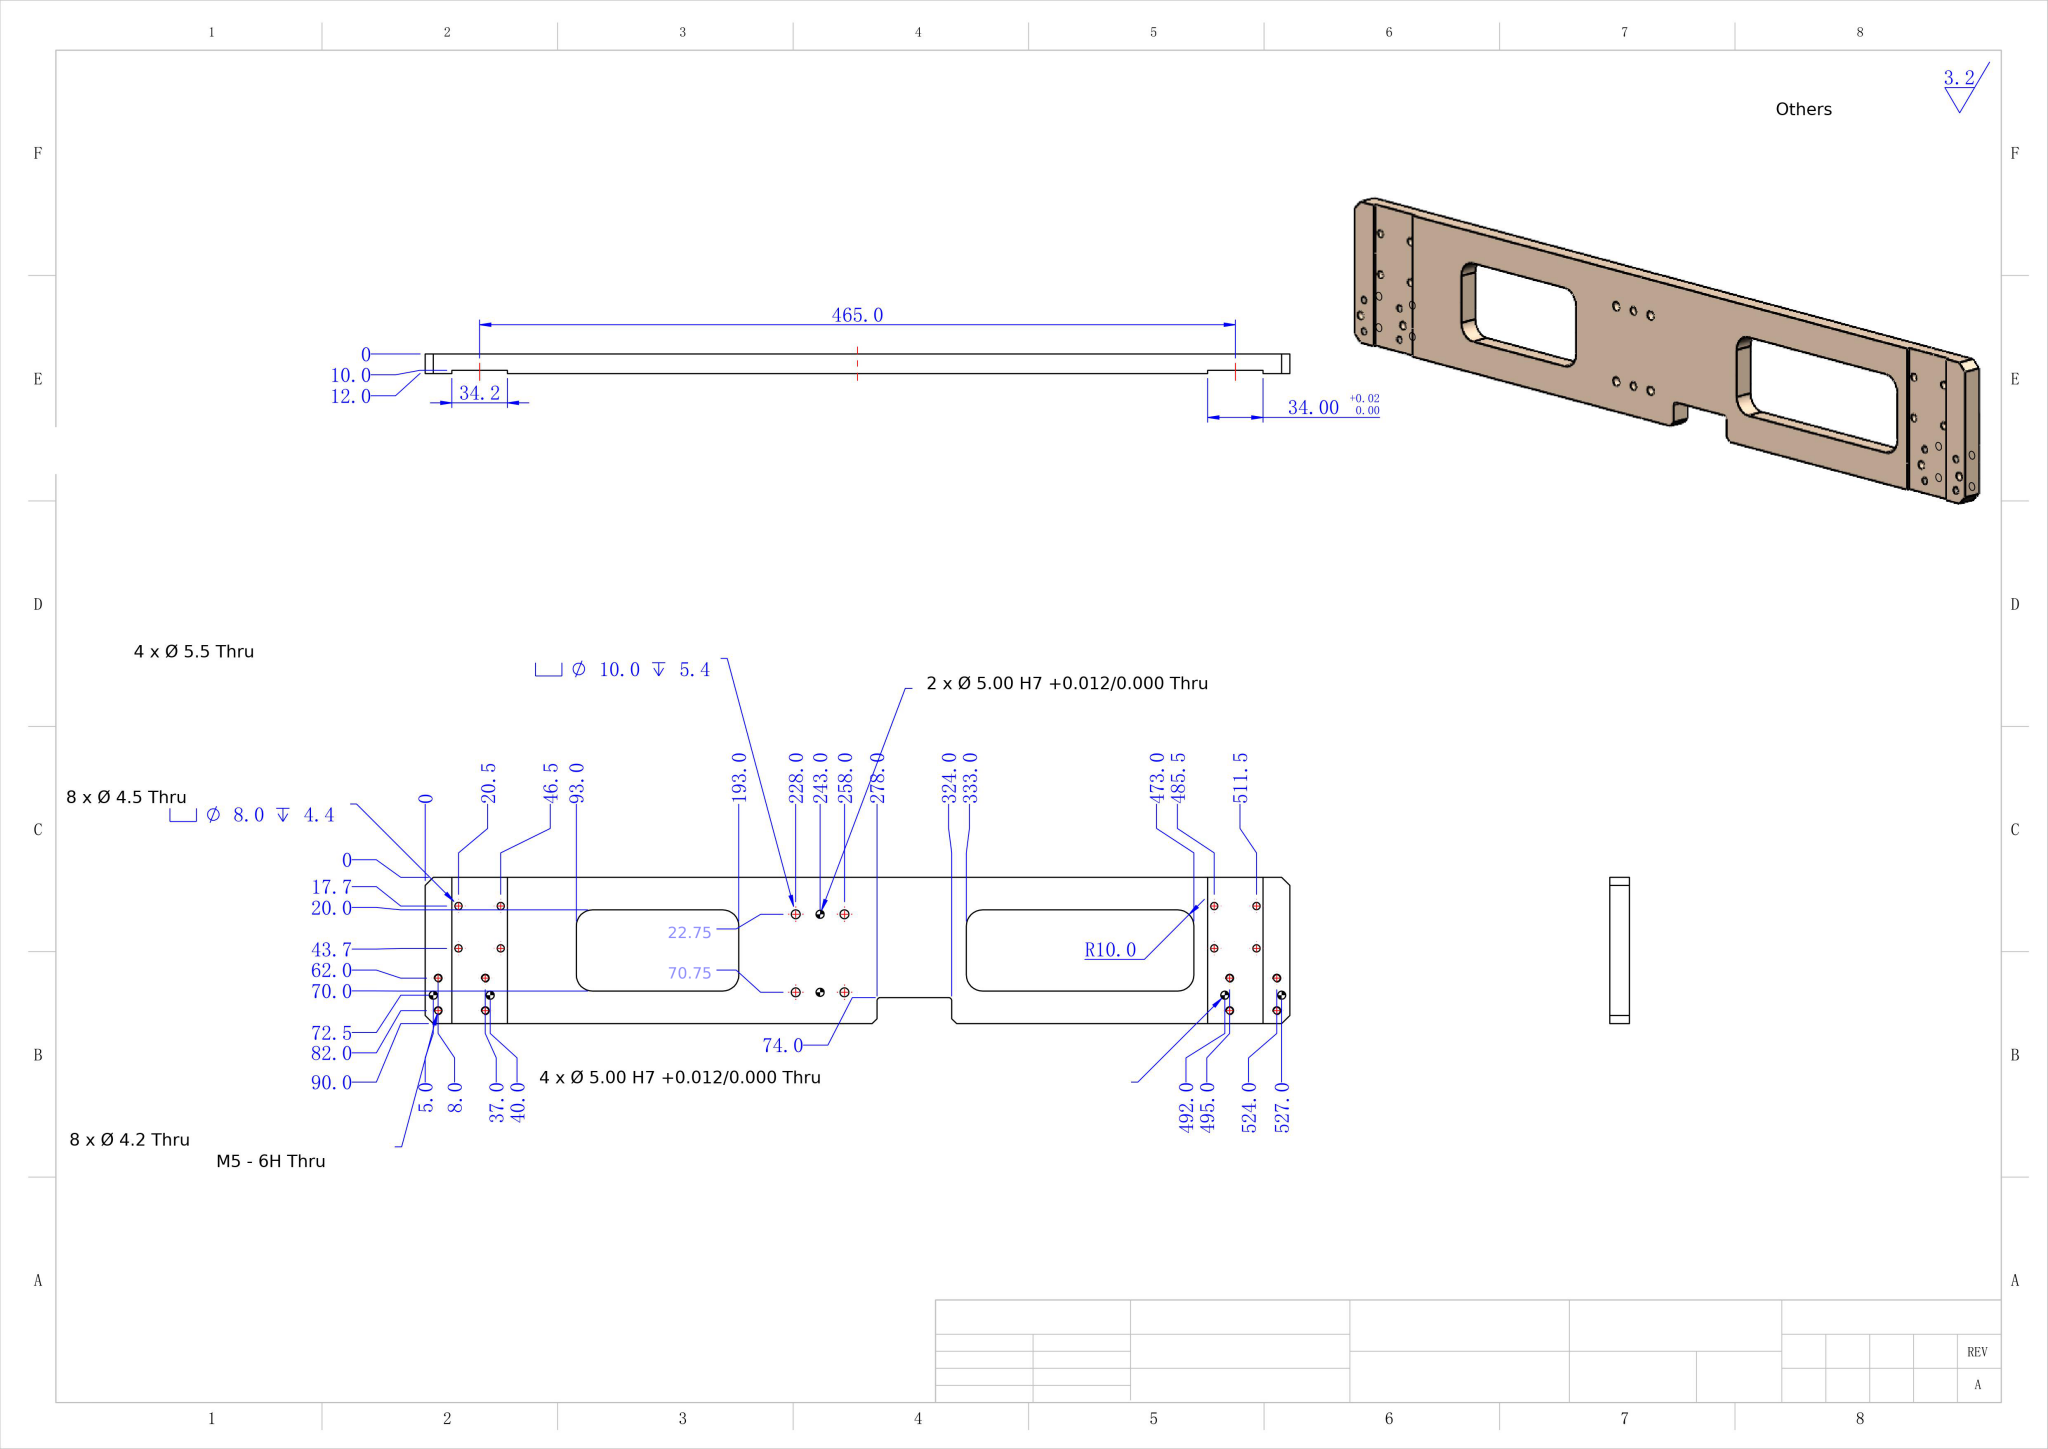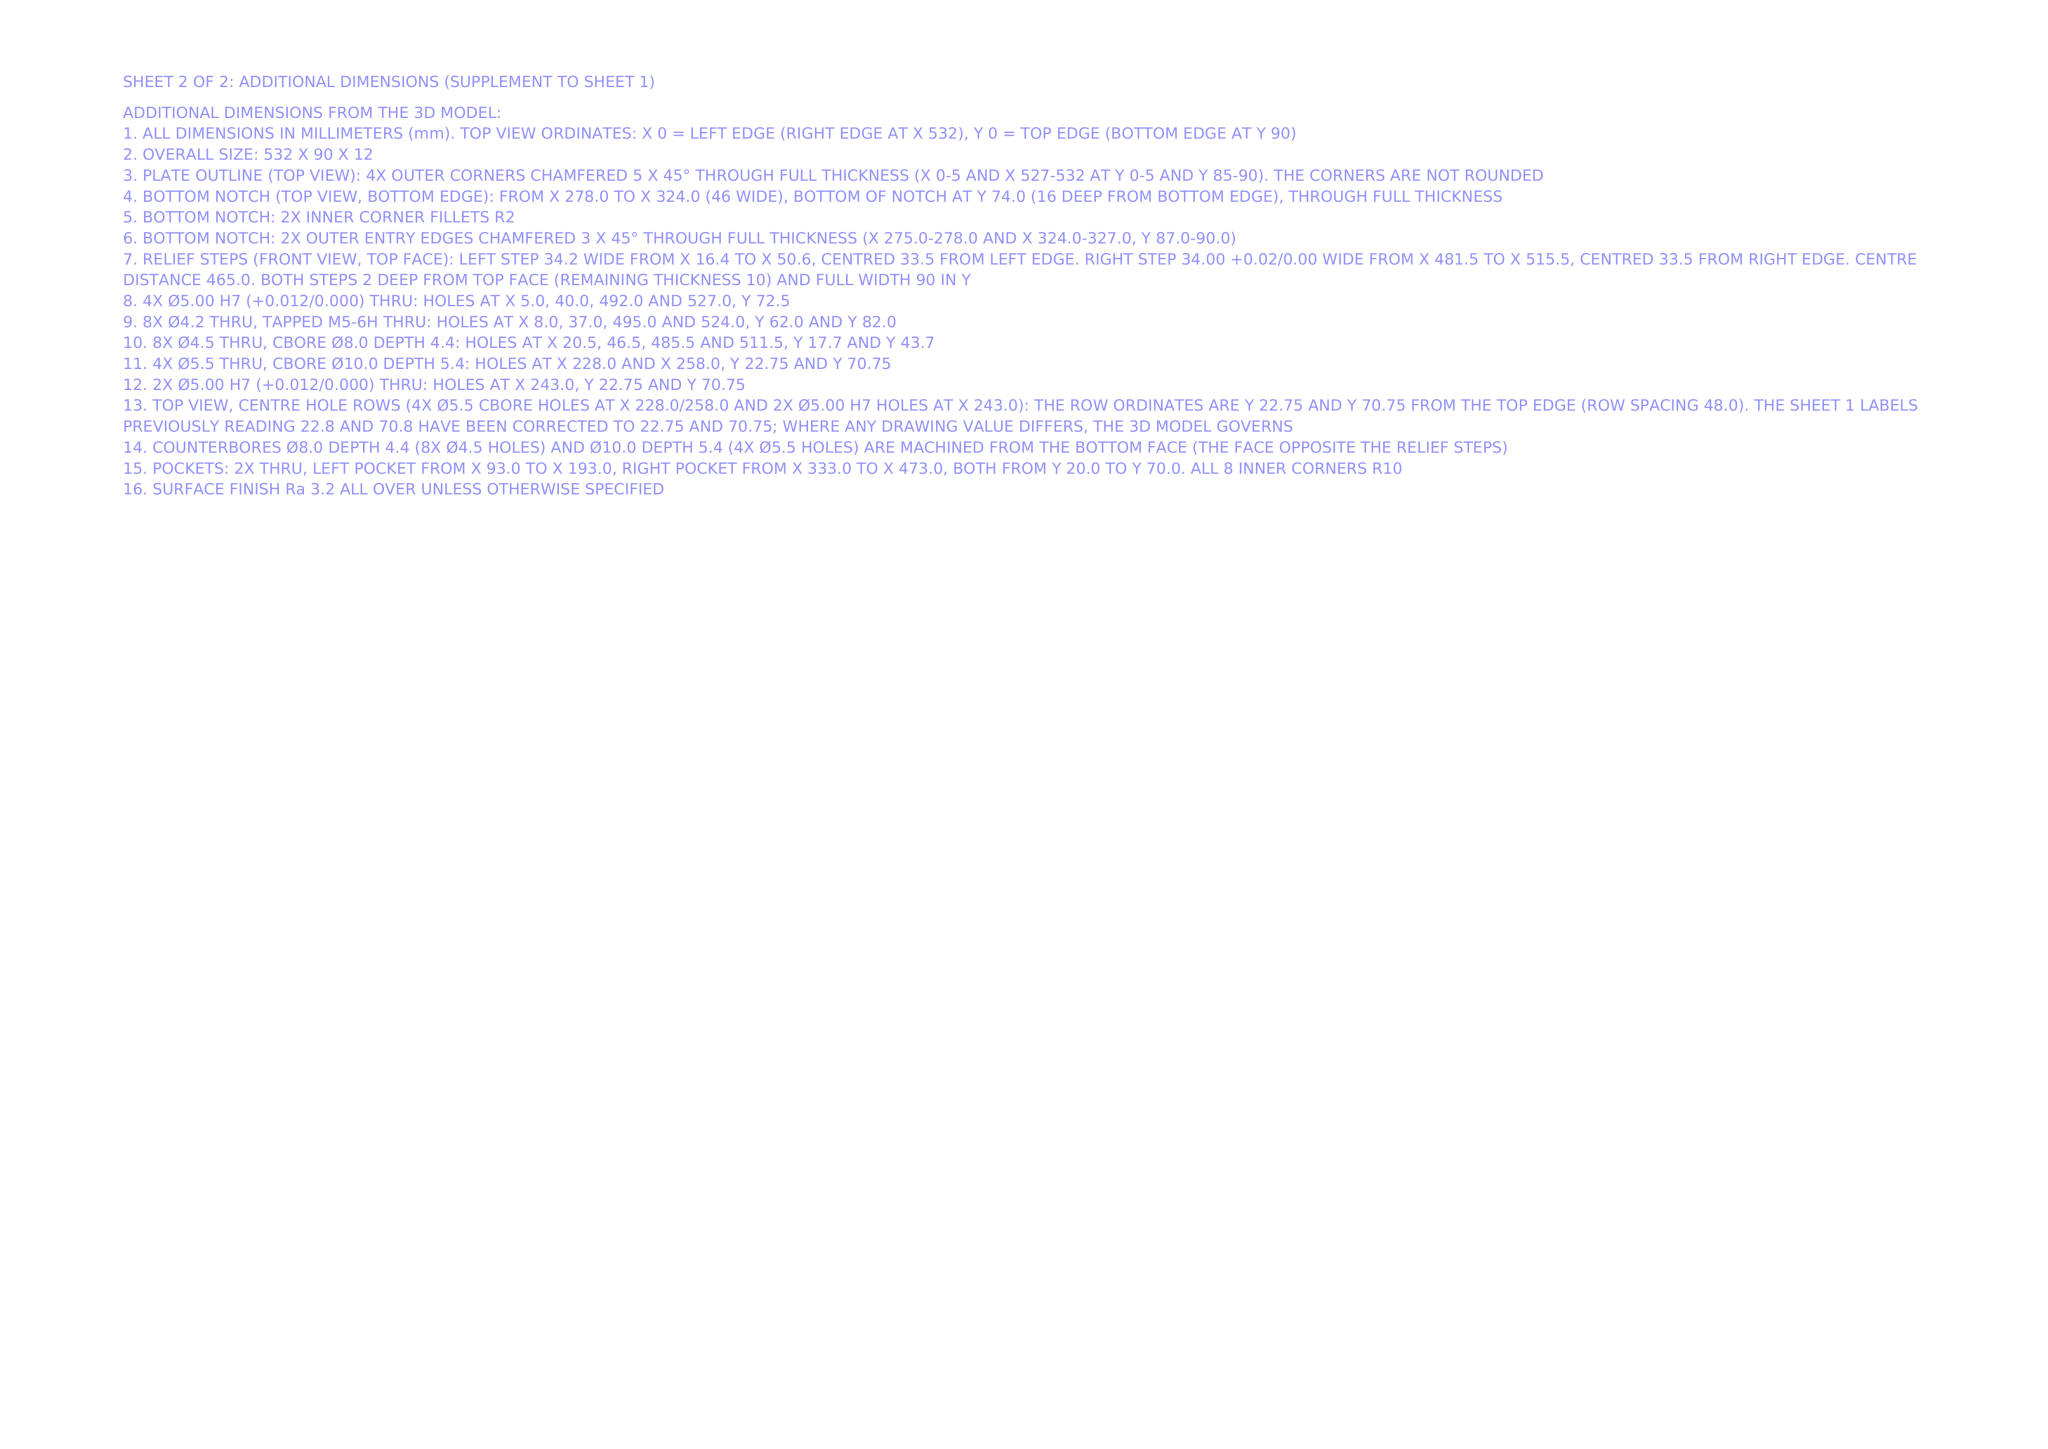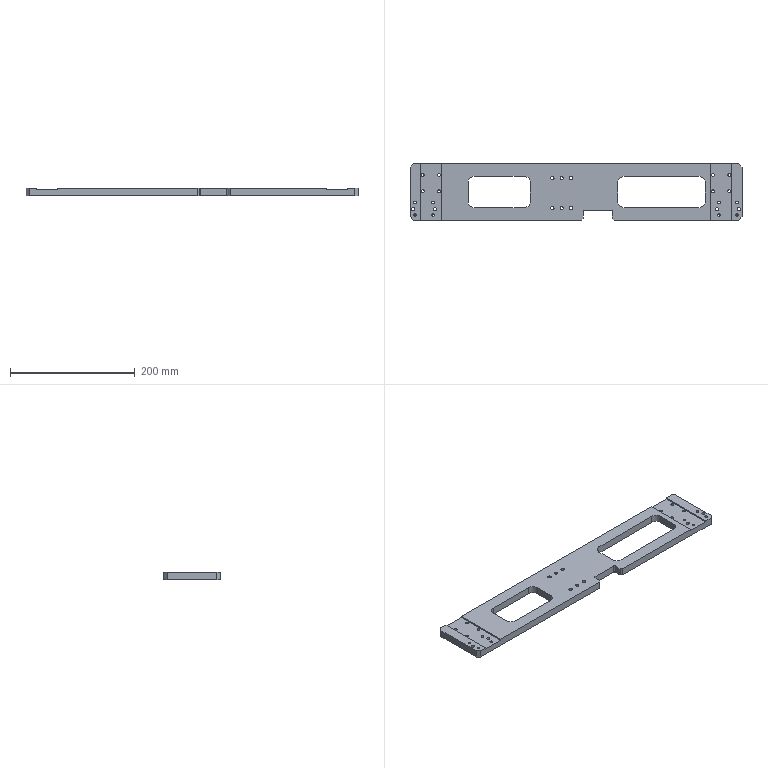Part | NX | mm | 1 solid | 130 faces | box 532 x 90 x 12 mm | volume 403465 mm3 | cylinder 86 | plane 44 | commonest cylinder face diameters 8 x16 4.5 x16 4.2 x16 5 x12 10 x8 5.5 x8 20 x8 4 x2